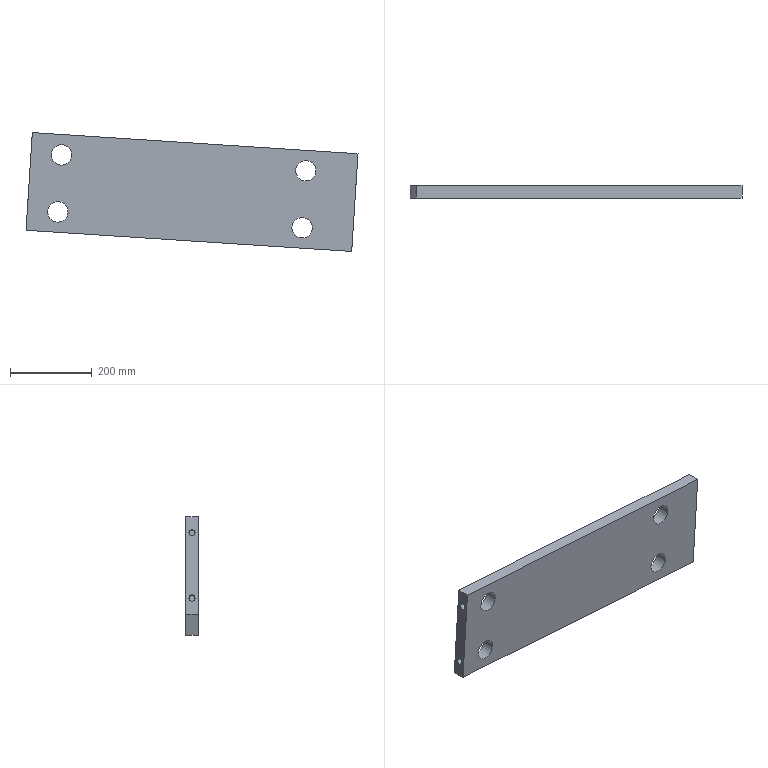Component | SolidWorks | X-AxisPedestal2-3 | 1 solid | 26 faces | box 813.86 x 30 x 291.29 mm | volume 5510243 mm3 | cylinder 16 | plane 10 | commonest cylinder face diameters 15 x8 50 x8
build123d program:
from build123d import *

# Parameters (mm, degrees)
SKETCH1_W               = 800
SKETCH1_H               = 240
BOSS_EXTRUDE1_DEPTH     = 30
CUT_EXTRUDE1_DEPTH      = 887.275
CUT_EXTRUDE1_DEPTH_BACK = 887.275
SKETCH2_R               = 25
SKETCH3_3_R             = 7.5
CUT_EXTRUDE2_DEPTH      = 20
CUT_EXTRUDE3_START      = -780
SKETCH3_3_2_R           = 7.5
CUT_EXTRUDE3_DEPTH      = 20


with BuildPart() as part:
    # Sketch1 → Boss-Extrude1 (new body)
    with BuildSketch(Plane.XY):
        with Locations((-153.487, 571.546)):
            Rectangle(SKETCH1_W, SKETCH1_H)
    extrude(amount=BOSS_EXTRUDE1_DEPTH)

    # Sketch2 → Cut-Extrude1 (cut, two sides: drawn at the far end of the back side and taken through both)
    with BuildSketch(Plane(origin=(0, 0, 0), x_dir=(-1, 0, 0), z_dir=(0, 0, -1)).offset(-CUT_EXTRUDE1_DEPTH_BACK)):
        with Locations((428.487, 501.546)):
            Circle(SKETCH2_R)
        with Locations((428.487, 641.546)):
            Circle(SKETCH2_R)
        with Locations((-171.513, 641.546)):
            Circle(SKETCH2_R)
        with Locations((-171.513, 501.546)):
            Circle(SKETCH2_R)
    extrude(amount=CUT_EXTRUDE1_DEPTH + CUT_EXTRUDE1_DEPTH_BACK, mode=Mode.SUBTRACT)

    # Sketch3_3 → Cut-Extrude2 (cut)
    with BuildSketch(Plane.ZY.offset(553.487)):
        with Locations((15, 651.546)):
            Circle(SKETCH3_3_R)
        with Locations((15, 491.546)):
            Circle(SKETCH3_3_R)
    extrude(amount=-CUT_EXTRUDE2_DEPTH, mode=Mode.SUBTRACT)

    # Sketch3_3 2 → Cut-Extrude3 (cut)
    with BuildSketch(Plane.ZY.offset(553.487).offset(CUT_EXTRUDE3_START)):
        with Locations((15, 651.546)):
            Circle(SKETCH3_3_2_R)
        with Locations((15, 491.546)):
            Circle(SKETCH3_3_2_R)
    extrude(amount=-CUT_EXTRUDE3_DEPTH, mode=Mode.SUBTRACT)


solid = part.part

# Placed as in the assembly
solid = solid.moved(Location((-106.284, -801, 289.801), (90, 0, 176.288)))
STEP:
#1=CARTESIAN_POINT('',(-14.744,-31.831,-13.611));
#2=VERTEX_POINT('',#1);
#3=CARTESIAN_POINT('',(-14.744,-32.421,-13.611));
#4=VERTEX_POINT('',#3);
#5=CARTESIAN_POINT('',(-14.744,-32.126,-13.611));
#6=DIRECTION('',(0.9979,0.,-0.06474));
#7=DIRECTION('',(0.06474,0.,0.9979));
#8=AXIS2_PLACEMENT_3D('',#5,#6,#7);
#9=CIRCLE('',#8,0.2953);
#10=EDGE_CURVE('',#2,#4,#9,.T.);
#11=ORIENTED_EDGE('',*,*,#10,.T.);
#12=CARTESIAN_POINT('',(-15.53,-32.421,-13.56));
#13=VERTEX_POINT('',#12);
#14=CARTESIAN_POINT('',(-14.744,-32.421,-13.611));
#15=DIRECTION('',(-0.9979,-0.,0.06474));
#16=VECTOR('',#15,39.37);
#17=LINE('',#14,#16);
#18=EDGE_CURVE('',#4,#13,#17,.T.);
#19=ORIENTED_EDGE('',*,*,#18,.T.);
#20=CARTESIAN_POINT('',(-15.53,-31.831,-13.56));
#21=VERTEX_POINT('',#20);
#22=CARTESIAN_POINT('',(-15.53,-32.126,-13.56));
#23=DIRECTION('',(0.9979,0.,-0.06474));
#24=DIRECTION('',(0.06474,0.,0.9979));
#25=AXIS2_PLACEMENT_3D('',#22,#23,#24);
#26=CIRCLE('',#25,0.2953);
#27=EDGE_CURVE('',#21,#13,#26,.T.);
#28=ORIENTED_EDGE('',*,*,#27,.F.);
#29=CARTESIAN_POINT('',(-14.744,-31.831,-13.611));
#30=DIRECTION('',(-0.9979,-0.,0.06474));
#31=VECTOR('',#30,39.37);
#32=LINE('',#29,#31);
#33=EDGE_CURVE('',#2,#21,#32,.T.);
#34=ORIENTED_EDGE('',*,*,#33,.F.);
#35=EDGE_LOOP('',(#11,#19,#28,#34));
#36=FACE_OUTER_BOUND('',#35,.T.);
#37=CARTESIAN_POINT('',(-14.744,-32.126,-13.611));
#38=DIRECTION('',(-0.9979,-0.,0.06474));
#39=DIRECTION('',(0.,1.,0.));
#40=AXIS2_PLACEMENT_3D('',#37,#38,#39);
#41=CYLINDRICAL_SURFACE('',#40,0.2953);
#42=ADVANCED_FACE('',(#36),#41,.F.);
#43=CARTESIAN_POINT('',(-14.336,-31.831,-7.325));
#44=VERTEX_POINT('',#43);
#45=CARTESIAN_POINT('',(-14.336,-32.421,-7.325));
#46=VERTEX_POINT('',#45);
#47=CARTESIAN_POINT('',(-14.336,-32.126,-7.325));
#48=DIRECTION('',(0.9979,0.,-0.06474));
#49=DIRECTION('',(0.06474,0.,0.9979));
#50=AXIS2_PLACEMENT_3D('',#47,#48,#49);
#51=CIRCLE('',#50,0.2953);
#52=EDGE_CURVE('',#44,#46,#51,.T.);
#53=ORIENTED_EDGE('',*,*,#52,.T.);
#54=CARTESIAN_POINT('',(-15.122,-32.421,-7.274));
#55=VERTEX_POINT('',#54);
#56=CARTESIAN_POINT('',(-14.336,-32.421,-7.325));
#57=DIRECTION('',(-0.9979,-0.,0.06474));
#58=VECTOR('',#57,39.37);
#59=LINE('',#56,#58);
#60=EDGE_CURVE('',#46,#55,#59,.T.);
#61=ORIENTED_EDGE('',*,*,#60,.T.);
#62=CARTESIAN_POINT('',(-15.122,-31.831,-7.274));
#63=VERTEX_POINT('',#62);
#64=CARTESIAN_POINT('',(-15.122,-32.126,-7.274));
#65=DIRECTION('',(0.9979,0.,-0.06474));
#66=DIRECTION('',(0.06474,0.,0.9979));
#67=AXIS2_PLACEMENT_3D('',#64,#65,#66);
#68=CIRCLE('',#67,0.2953);
#69=EDGE_CURVE('',#63,#55,#68,.T.);
#70=ORIENTED_EDGE('',*,*,#69,.F.);
#71=CARTESIAN_POINT('',(-14.336,-31.831,-7.325));
#72=DIRECTION('',(-0.9979,-0.,0.06474));
#73=VECTOR('',#72,39.37);
#74=LINE('',#71,#73);
#75=EDGE_CURVE('',#44,#63,#74,.T.);
#76=ORIENTED_EDGE('',*,*,#75,.F.);
#77=EDGE_LOOP('',(#53,#61,#70,#76));
#78=FACE_OUTER_BOUND('',#77,.T.);
#79=CARTESIAN_POINT('',(-14.336,-32.126,-7.325));
#80=DIRECTION('',(-0.9979,-0.,0.06474));
#81=DIRECTION('',(0.,1.,0.));
#82=AXIS2_PLACEMENT_3D('',#79,#80,#81);
#83=CYLINDRICAL_SURFACE('',#82,0.2953);
#84=ADVANCED_FACE('',(#78),#83,.F.);
#85=CARTESIAN_POINT('',(15.522,-31.831,-9.262));
#86=VERTEX_POINT('',#85);
#87=CARTESIAN_POINT('',(15.522,-32.421,-9.262));
#88=VERTEX_POINT('',#87);
#89=CARTESIAN_POINT('',(15.522,-32.126,-9.262));
#90=DIRECTION('',(0.9979,0.,-0.06474));
#91=DIRECTION('',(0.,-1.,0.));
#92=AXIS2_PLACEMENT_3D('',#89,#90,#91);
#93=CIRCLE('',#92,0.2953);
#94=EDGE_CURVE('',#86,#88,#93,.T.);
#95=ORIENTED_EDGE('',*,*,#94,.F.);
#96=CARTESIAN_POINT('',(16.308,-31.831,-9.313));
#97=VERTEX_POINT('',#96);
#98=CARTESIAN_POINT('',(15.522,-31.831,-9.262));
#99=DIRECTION('',(0.9979,0.,-0.06474));
#100=VECTOR('',#99,39.37);
#101=LINE('',#98,#100);
#102=EDGE_CURVE('',#86,#97,#101,.T.);
#103=ORIENTED_EDGE('',*,*,#102,.T.);
#104=CARTESIAN_POINT('',(16.308,-32.421,-9.313));
#105=VERTEX_POINT('',#104);
#106=CARTESIAN_POINT('',(16.308,-32.126,-9.313));
#107=DIRECTION('',(0.9979,0.,-0.06474));
#108=DIRECTION('',(0.,-1.,0.));
#109=AXIS2_PLACEMENT_3D('',#106,#107,#108);
#110=CIRCLE('',#109,0.2953);
#111=EDGE_CURVE('',#97,#105,#110,.T.);
#112=ORIENTED_EDGE('',*,*,#111,.T.);
#113=CARTESIAN_POINT('',(15.522,-32.421,-9.262));
#114=DIRECTION('',(0.9979,0.,-0.06474));
#115=VECTOR('',#114,39.37);
#116=LINE('',#113,#115);
#117=EDGE_CURVE('',#88,#105,#116,.T.);
#118=ORIENTED_EDGE('',*,*,#117,.F.);
#119=EDGE_LOOP('',(#95,#103,#112,#118));
#120=FACE_OUTER_BOUND('',#119,.T.);
#121=CARTESIAN_POINT('',(15.522,-32.126,-9.262));
#122=DIRECTION('',(0.9979,0.,-0.06474));
#123=DIRECTION('',(0.,-1.,0.));
#124=AXIS2_PLACEMENT_3D('',#121,#122,#123);
#125=CYLINDRICAL_SURFACE('',#124,0.2953);
#126=ADVANCED_FACE('',(#120),#125,.F.);
#127=CARTESIAN_POINT('',(15.114,-31.831,-15.548));
#128=VERTEX_POINT('',#127);
#129=CARTESIAN_POINT('',(15.114,-32.421,-15.548));
#130=VERTEX_POINT('',#129);
#131=CARTESIAN_POINT('',(15.114,-32.126,-15.548));
#132=DIRECTION('',(0.9979,0.,-0.06474));
#133=DIRECTION('',(0.,-1.,0.));
#134=AXIS2_PLACEMENT_3D('',#131,#132,#133);
#135=CIRCLE('',#134,0.2953);
#136=EDGE_CURVE('',#128,#130,#135,.T.);
#137=ORIENTED_EDGE('',*,*,#136,.F.);
#138=CARTESIAN_POINT('',(15.9,-31.831,-15.599));
#139=VERTEX_POINT('',#138);
#140=CARTESIAN_POINT('',(15.114,-31.831,-15.548));
#141=DIRECTION('',(0.9979,0.,-0.06474));
#142=VECTOR('',#141,39.37);
#143=LINE('',#140,#142);
#144=EDGE_CURVE('',#128,#139,#143,.T.);
#145=ORIENTED_EDGE('',*,*,#144,.T.);
#146=CARTESIAN_POINT('',(15.9,-32.421,-15.599));
#147=VERTEX_POINT('',#146);
#148=CARTESIAN_POINT('',(15.9,-32.126,-15.599));
#149=DIRECTION('',(0.9979,0.,-0.06474));
#150=DIRECTION('',(0.,-1.,0.));
#151=AXIS2_PLACEMENT_3D('',#148,#149,#150);
#152=CIRCLE('',#151,0.2953);
#153=EDGE_CURVE('',#139,#147,#152,.T.);
#154=ORIENTED_EDGE('',*,*,#153,.T.);
#155=CARTESIAN_POINT('',(15.114,-32.421,-15.548));
#156=DIRECTION('',(0.9979,0.,-0.06474));
#157=VECTOR('',#156,39.37);
#158=LINE('',#155,#157);
#159=EDGE_CURVE('',#130,#147,#158,.T.);
#160=ORIENTED_EDGE('',*,*,#159,.F.);
#161=EDGE_LOOP('',(#137,#145,#154,#160));
#162=FACE_OUTER_BOUND('',#161,.T.);
#163=CARTESIAN_POINT('',(15.114,-32.126,-15.548));
#164=DIRECTION('',(0.9979,0.,-0.06474));
#165=DIRECTION('',(0.,-1.,0.));
#166=AXIS2_PLACEMENT_3D('',#163,#164,#165);
#167=CYLINDRICAL_SURFACE('',#166,0.2953);
#168=ADVANCED_FACE('',(#162),#167,.F.);
#169=CARTESIAN_POINT('',(-13.183,-32.717,-7.794));
#170=VERTEX_POINT('',#169);
#171=CARTESIAN_POINT('',(-11.219,-32.717,-7.922));
#172=VERTEX_POINT('',#171);
#173=CARTESIAN_POINT('',(-12.201,-32.717,-7.858));
#174=DIRECTION('',(-0.,1.,0.));
#175=DIRECTION('',(0.9979,0.,-0.06474));
#176=AXIS2_PLACEMENT_3D('',#173,#174,#175);
#177=CIRCLE('',#176,0.9843);
#178=EDGE_CURVE('',#170,#172,#177,.T.);
#179=ORIENTED_EDGE('',*,*,#178,.F.);
#180=CARTESIAN_POINT('',(-13.183,-31.535,-7.794));
#181=VERTEX_POINT('',#180);
#182=CARTESIAN_POINT('',(-13.183,-32.717,-7.794));
#183=DIRECTION('',(-0.,1.,0.));
#184=VECTOR('',#183,39.37);
#185=LINE('',#182,#184);
#186=EDGE_CURVE('',#170,#181,#185,.T.);
#187=ORIENTED_EDGE('',*,*,#186,.T.);
#188=CARTESIAN_POINT('',(-11.219,-31.535,-7.922));
#189=VERTEX_POINT('',#188);
#190=CARTESIAN_POINT('',(-12.201,-31.535,-7.858));
#191=DIRECTION('',(-0.,1.,0.));
#192=DIRECTION('',(0.9979,0.,-0.06474));
#193=AXIS2_PLACEMENT_3D('',#190,#191,#192);
#194=CIRCLE('',#193,0.9843);
#195=EDGE_CURVE('',#181,#189,#194,.T.);
#196=ORIENTED_EDGE('',*,*,#195,.T.);
#197=CARTESIAN_POINT('',(-11.219,-32.717,-7.922));
#198=DIRECTION('',(-0.,1.,0.));
#199=VECTOR('',#198,39.37);
#200=LINE('',#197,#199);
#201=EDGE_CURVE('',#172,#189,#200,.T.);
#202=ORIENTED_EDGE('',*,*,#201,.F.);
#203=EDGE_LOOP('',(#179,#187,#196,#202));
#204=FACE_OUTER_BOUND('',#203,.T.);
#205=CARTESIAN_POINT('',(-12.201,-32.717,-7.858));
#206=DIRECTION('',(-0.,1.,0.));
#207=DIRECTION('',(0.9979,0.,-0.06474));
#208=AXIS2_PLACEMENT_3D('',#205,#206,#207);
#209=CYLINDRICAL_SURFACE('',#208,0.9843);
#210=ADVANCED_FACE('',(#204),#209,.F.);
#211=CARTESIAN_POINT('',(-13.54,-32.717,-13.294));
#212=VERTEX_POINT('',#211);
#213=CARTESIAN_POINT('',(-11.576,-32.717,-13.422));
#214=VERTEX_POINT('',#213);
#215=CARTESIAN_POINT('',(-12.558,-32.717,-13.358));
#216=DIRECTION('',(-0.,1.,0.));
#217=DIRECTION('',(0.9979,0.,-0.06474));
#218=AXIS2_PLACEMENT_3D('',#215,#216,#217);
#219=CIRCLE('',#218,0.9843);
#220=EDGE_CURVE('',#212,#214,#219,.T.);
#221=ORIENTED_EDGE('',*,*,#220,.F.);
#222=CARTESIAN_POINT('',(-13.54,-31.535,-13.294));
#223=VERTEX_POINT('',#222);
#224=CARTESIAN_POINT('',(-13.54,-32.717,-13.294));
#225=DIRECTION('',(-0.,1.,0.));
#226=VECTOR('',#225,39.37);
#227=LINE('',#224,#226);
#228=EDGE_CURVE('',#212,#223,#227,.T.);
#229=ORIENTED_EDGE('',*,*,#228,.T.);
#230=CARTESIAN_POINT('',(-11.576,-31.535,-13.422));
#231=VERTEX_POINT('',#230);
#232=CARTESIAN_POINT('',(-12.558,-31.535,-13.358));
#233=DIRECTION('',(-0.,1.,0.));
#234=DIRECTION('',(0.9979,0.,-0.06474));
#235=AXIS2_PLACEMENT_3D('',#232,#233,#234);
#236=CIRCLE('',#235,0.9843);
#237=EDGE_CURVE('',#223,#231,#236,.T.);
#238=ORIENTED_EDGE('',*,*,#237,.T.);
#239=CARTESIAN_POINT('',(-11.576,-32.717,-13.422));
#240=DIRECTION('',(-0.,1.,0.));
#241=VECTOR('',#240,39.37);
#242=LINE('',#239,#241);
#243=EDGE_CURVE('',#214,#231,#242,.T.);
#244=ORIENTED_EDGE('',*,*,#243,.F.);
#245=EDGE_LOOP('',(#221,#229,#238,#244));
#246=FACE_OUTER_BOUND('',#245,.T.);
#247=CARTESIAN_POINT('',(-12.558,-32.717,-13.358));
#248=DIRECTION('',(-0.,1.,0.));
#249=DIRECTION('',(0.9979,0.,-0.06474));
#250=AXIS2_PLACEMENT_3D('',#247,#248,#249);
#251=CYLINDRICAL_SURFACE('',#250,0.9843);
#252=ADVANCED_FACE('',(#246),#251,.F.);
#253=CARTESIAN_POINT('',(10.032,-32.717,-14.824));
#254=VERTEX_POINT('',#253);
#255=CARTESIAN_POINT('',(11.997,-32.717,-14.951));
#256=VERTEX_POINT('',#255);
#257=CARTESIAN_POINT('',(11.015,-32.717,-14.887));
#258=DIRECTION('',(-0.,1.,0.));
#259=DIRECTION('',(0.9979,0.,-0.06474));
#260=AXIS2_PLACEMENT_3D('',#257,#258,#259);
#261=CIRCLE('',#260,0.9843);
#262=EDGE_CURVE('',#254,#256,#261,.T.);
#263=ORIENTED_EDGE('',*,*,#262,.F.);
#264=CARTESIAN_POINT('',(10.032,-31.535,-14.824));
#265=VERTEX_POINT('',#264);
#266=CARTESIAN_POINT('',(10.032,-32.717,-14.824));
#267=DIRECTION('',(-0.,1.,0.));
#268=VECTOR('',#267,39.37);
#269=LINE('',#266,#268);
#270=EDGE_CURVE('',#254,#265,#269,.T.);
#271=ORIENTED_EDGE('',*,*,#270,.T.);
#272=CARTESIAN_POINT('',(11.997,-31.535,-14.951));
#273=VERTEX_POINT('',#272);
#274=CARTESIAN_POINT('',(11.015,-31.535,-14.887));
#275=DIRECTION('',(-0.,1.,0.));
#276=DIRECTION('',(0.9979,0.,-0.06474));
#277=AXIS2_PLACEMENT_3D('',#274,#275,#276);
#278=CIRCLE('',#277,0.9843);
#279=EDGE_CURVE('',#265,#273,#278,.T.);
#280=ORIENTED_EDGE('',*,*,#279,.T.);
#281=CARTESIAN_POINT('',(11.997,-32.717,-14.951));
#282=DIRECTION('',(-0.,1.,0.));
#283=VECTOR('',#282,39.37);
#284=LINE('',#281,#283);
#285=EDGE_CURVE('',#256,#273,#284,.T.);
#286=ORIENTED_EDGE('',*,*,#285,.F.);
#287=EDGE_LOOP('',(#263,#271,#280,#286));
#288=FACE_OUTER_BOUND('',#287,.T.);
#289=CARTESIAN_POINT('',(11.015,-32.717,-14.887));
#290=DIRECTION('',(-0.,1.,0.));
#291=DIRECTION('',(0.9979,0.,-0.06474));
#292=AXIS2_PLACEMENT_3D('',#289,#290,#291);
#293=CYLINDRICAL_SURFACE('',#292,0.9843);
#294=ADVANCED_FACE('',(#288),#293,.F.);
#295=CARTESIAN_POINT('',(10.389,-32.717,-9.323));
#296=VERTEX_POINT('',#295);
#297=CARTESIAN_POINT('',(12.354,-32.717,-9.451));
#298=VERTEX_POINT('',#297);
#299=CARTESIAN_POINT('',(11.371,-32.717,-9.387));
#300=DIRECTION('',(-0.,1.,0.));
#301=DIRECTION('',(0.9979,0.,-0.06474));
#302=AXIS2_PLACEMENT_3D('',#299,#300,#301);
#303=CIRCLE('',#302,0.9843);
#304=EDGE_CURVE('',#296,#298,#303,.T.);
#305=ORIENTED_EDGE('',*,*,#304,.F.);
#306=CARTESIAN_POINT('',(10.389,-31.535,-9.323));
#307=VERTEX_POINT('',#306);
#308=CARTESIAN_POINT('',(10.389,-32.717,-9.323));
#309=DIRECTION('',(-0.,1.,0.));
#310=VECTOR('',#309,39.37);
#311=LINE('',#308,#310);
#312=EDGE_CURVE('',#296,#307,#311,.T.);
#313=ORIENTED_EDGE('',*,*,#312,.T.);
#314=CARTESIAN_POINT('',(12.354,-31.535,-9.451));
#315=VERTEX_POINT('',#314);
#316=CARTESIAN_POINT('',(11.371,-31.535,-9.387));
#317=DIRECTION('',(-0.,1.,0.));
#318=DIRECTION('',(0.9979,0.,-0.06474));
#319=AXIS2_PLACEMENT_3D('',#316,#317,#318);
#320=CIRCLE('',#319,0.9843);
#321=EDGE_CURVE('',#307,#315,#320,.T.);
#322=ORIENTED_EDGE('',*,*,#321,.T.);
#323=CARTESIAN_POINT('',(12.354,-32.717,-9.451));
#324=DIRECTION('',(-0.,1.,0.));
#325=VECTOR('',#324,39.37);
#326=LINE('',#323,#325);
#327=EDGE_CURVE('',#298,#315,#326,.T.);
#328=ORIENTED_EDGE('',*,*,#327,.F.);
#329=EDGE_LOOP('',(#305,#313,#322,#328));
#330=FACE_OUTER_BOUND('',#329,.T.);
#331=CARTESIAN_POINT('',(11.371,-32.717,-9.387));
#332=DIRECTION('',(-0.,1.,0.));
#333=DIRECTION('',(0.9979,0.,-0.06474));
#334=AXIS2_PLACEMENT_3D('',#331,#332,#333);
#335=CYLINDRICAL_SURFACE('',#334,0.9843);
#336=ADVANCED_FACE('',(#330),#335,.F.);
#337=ORIENTED_EDGE('',*,*,#27,.T.);
#338=CARTESIAN_POINT('',(-15.53,-32.126,-13.56));
#339=DIRECTION('',(0.9979,0.,-0.06474));
#340=DIRECTION('',(0.06474,0.,0.9979));
#341=AXIS2_PLACEMENT_3D('',#338,#339,#340);
#342=CIRCLE('',#341,0.2953);
#343=EDGE_CURVE('',#13,#21,#342,.T.);
#344=ORIENTED_EDGE('',*,*,#343,.T.);
#345=EDGE_LOOP('',(#337,#344));
#346=FACE_BOUND('',#345,.T.);
#347=ORIENTED_EDGE('',*,*,#69,.T.);
#348=CARTESIAN_POINT('',(-15.122,-32.126,-7.274));
#349=DIRECTION('',(0.9979,0.,-0.06474));
#350=DIRECTION('',(0.06474,0.,0.9979));
#351=AXIS2_PLACEMENT_3D('',#348,#349,#350);
#352=CIRCLE('',#351,0.2953);
#353=EDGE_CURVE('',#55,#63,#352,.T.);
#354=ORIENTED_EDGE('',*,*,#353,.T.);
#355=EDGE_LOOP('',(#347,#354));
#356=FACE_BOUND('',#355,.T.);
#357=CARTESIAN_POINT('',(-15.02,-31.535,-5.702));
#358=VERTEX_POINT('',#357);
#359=CARTESIAN_POINT('',(-15.632,-31.535,-15.131));
#360=VERTEX_POINT('',#359);
#361=CARTESIAN_POINT('',(-15.632,-31.535,-15.131));
#362=DIRECTION('',(-0.06474,0.,-0.9979));
#363=VECTOR('',#362,39.37);
#364=LINE('',#361,#363);
#365=EDGE_CURVE('',#358,#360,#364,.T.);
#366=ORIENTED_EDGE('',*,*,#365,.T.);
#367=CARTESIAN_POINT('',(-15.632,-32.717,-15.131));
#368=VERTEX_POINT('',#367);
#369=CARTESIAN_POINT('',(-15.632,-32.717,-15.131));
#370=DIRECTION('',(-0.,1.,0.));
#371=VECTOR('',#370,39.37);
#372=LINE('',#369,#371);
#373=EDGE_CURVE('',#368,#360,#372,.T.);
#374=ORIENTED_EDGE('',*,*,#373,.F.);
#375=CARTESIAN_POINT('',(-15.02,-32.717,-5.702));
#376=VERTEX_POINT('',#375);
#377=CARTESIAN_POINT('',(-15.632,-32.717,-15.131));
#378=DIRECTION('',(-0.06474,0.,-0.9979));
#379=VECTOR('',#378,39.37);
#380=LINE('',#377,#379);
#381=EDGE_CURVE('',#376,#368,#380,.T.);
#382=ORIENTED_EDGE('',*,*,#381,.F.);
#383=CARTESIAN_POINT('',(-15.02,-32.717,-5.702));
#384=DIRECTION('',(-0.,1.,0.));
#385=VECTOR('',#384,39.37);
#386=LINE('',#383,#385);
#387=EDGE_CURVE('',#376,#358,#386,.T.);
#388=ORIENTED_EDGE('',*,*,#387,.T.);
#389=EDGE_LOOP('',(#366,#374,#382,#388));
#390=FACE_OUTER_BOUND('',#389,.T.);
#391=CARTESIAN_POINT('',(-15.632,-32.717,-15.131));
#392=DIRECTION('',(0.9979,0.,-0.06474));
#393=DIRECTION('',(0.06474,-0.,0.9979));
#394=AXIS2_PLACEMENT_3D('',#391,#392,#393);
#395=PLANE('',#394);
#396=ADVANCED_FACE('',(#346,#356,#390),#395,.F.);
#397=CARTESIAN_POINT('',(15.798,-31.535,-17.17));
#398=VERTEX_POINT('',#397);
#399=CARTESIAN_POINT('',(-15.632,-31.535,-15.131));
#400=DIRECTION('',(0.9979,0.,-0.06474));
#401=VECTOR('',#400,39.37);
#402=LINE('',#399,#401);
#403=EDGE_CURVE('',#360,#398,#402,.T.);
#404=ORIENTED_EDGE('',*,*,#403,.T.);
#405=CARTESIAN_POINT('',(15.798,-32.717,-17.17));
#406=VERTEX_POINT('',#405);
#407=CARTESIAN_POINT('',(15.798,-32.717,-17.17));
#408=DIRECTION('',(-0.,1.,0.));
#409=VECTOR('',#408,39.37);
#410=LINE('',#407,#409);
#411=EDGE_CURVE('',#406,#398,#410,.T.);
#412=ORIENTED_EDGE('',*,*,#411,.F.);
#413=CARTESIAN_POINT('',(-15.632,-32.717,-15.131));
#414=DIRECTION('',(0.9979,0.,-0.06474));
#415=VECTOR('',#414,39.37);
#416=LINE('',#413,#415);
#417=EDGE_CURVE('',#368,#406,#416,.T.);
#418=ORIENTED_EDGE('',*,*,#417,.F.);
#419=ORIENTED_EDGE('',*,*,#373,.T.);
#420=EDGE_LOOP('',(#404,#412,#418,#419));
#421=FACE_OUTER_BOUND('',#420,.T.);
#422=CARTESIAN_POINT('',(-15.632,-32.717,-15.131));
#423=DIRECTION('',(0.06474,-0.,0.9979));
#424=DIRECTION('',(-0.9979,-0.,0.06474));
#425=AXIS2_PLACEMENT_3D('',#422,#423,#424);
#426=PLANE('',#425);
#427=ADVANCED_FACE('',(#421),#426,.F.);
#428=CARTESIAN_POINT('',(16.308,-32.126,-9.313));
#429=DIRECTION('',(0.9979,0.,-0.06474));
#430=DIRECTION('',(0.,-1.,0.));
#431=AXIS2_PLACEMENT_3D('',#428,#429,#430);
#432=CIRCLE('',#431,0.2953);
#433=EDGE_CURVE('',#105,#97,#432,.T.);
#434=ORIENTED_EDGE('',*,*,#433,.F.);
#435=ORIENTED_EDGE('',*,*,#111,.F.);
#436=EDGE_LOOP('',(#434,#435));
#437=FACE_BOUND('',#436,.T.);
#438=CARTESIAN_POINT('',(15.9,-32.126,-15.599));
#439=DIRECTION('',(0.9979,0.,-0.06474));
#440=DIRECTION('',(0.,-1.,0.));
#441=AXIS2_PLACEMENT_3D('',#438,#439,#440);
#442=CIRCLE('',#441,0.2953);
#443=EDGE_CURVE('',#147,#139,#442,.T.);
#444=ORIENTED_EDGE('',*,*,#443,.F.);
#445=ORIENTED_EDGE('',*,*,#153,.F.);
#446=EDGE_LOOP('',(#444,#445));
#447=FACE_BOUND('',#446,.T.);
#448=CARTESIAN_POINT('',(16.41,-31.535,-7.741));
#449=VERTEX_POINT('',#448);
#450=CARTESIAN_POINT('',(15.798,-31.535,-17.17));
#451=DIRECTION('',(0.06474,-0.,0.9979));
#452=VECTOR('',#451,39.37);
#453=LINE('',#450,#452);
#454=EDGE_CURVE('',#398,#449,#453,.T.);
#455=ORIENTED_EDGE('',*,*,#454,.T.);
#456=CARTESIAN_POINT('',(16.41,-32.717,-7.741));
#457=VERTEX_POINT('',#456);
#458=CARTESIAN_POINT('',(16.41,-32.717,-7.741));
#459=DIRECTION('',(-0.,1.,0.));
#460=VECTOR('',#459,39.37);
#461=LINE('',#458,#460);
#462=EDGE_CURVE('',#457,#449,#461,.T.);
#463=ORIENTED_EDGE('',*,*,#462,.F.);
#464=CARTESIAN_POINT('',(15.798,-32.717,-17.17));
#465=DIRECTION('',(0.06474,-0.,0.9979));
#466=VECTOR('',#465,39.37);
#467=LINE('',#464,#466);
#468=EDGE_CURVE('',#406,#457,#467,.T.);
#469=ORIENTED_EDGE('',*,*,#468,.F.);
#470=ORIENTED_EDGE('',*,*,#411,.T.);
#471=EDGE_LOOP('',(#455,#463,#469,#470));
#472=FACE_OUTER_BOUND('',#471,.T.);
#473=CARTESIAN_POINT('',(15.798,-32.717,-17.17));
#474=DIRECTION('',(-0.9979,-0.,0.06474));
#475=DIRECTION('',(-0.,1.,0.));
#476=AXIS2_PLACEMENT_3D('',#473,#474,#475);
#477=PLANE('',#476);
#478=ADVANCED_FACE('',(#437,#447,#472),#477,.F.);
#479=CARTESIAN_POINT('',(-15.02,-31.535,-5.702));
#480=DIRECTION('',(-0.9979,-0.,0.06474));
#481=VECTOR('',#480,39.37);
#482=LINE('',#479,#481);
#483=EDGE_CURVE('',#449,#358,#482,.T.);
#484=ORIENTED_EDGE('',*,*,#483,.T.);
#485=ORIENTED_EDGE('',*,*,#387,.F.);
#486=CARTESIAN_POINT('',(-15.02,-32.717,-5.702));
#487=DIRECTION('',(-0.9979,-0.,0.06474));
#488=VECTOR('',#487,39.37);
#489=LINE('',#486,#488);
#490=EDGE_CURVE('',#457,#376,#489,.T.);
#491=ORIENTED_EDGE('',*,*,#490,.F.);
#492=ORIENTED_EDGE('',*,*,#462,.T.);
#493=EDGE_LOOP('',(#484,#485,#491,#492));
#494=FACE_OUTER_BOUND('',#493,.T.);
#495=CARTESIAN_POINT('',(-15.02,-32.717,-5.702));
#496=DIRECTION('',(-0.06474,0.,-0.9979));
#497=DIRECTION('',(0.9979,0.,-0.06474));
#498=AXIS2_PLACEMENT_3D('',#495,#496,#497);
#499=PLANE('',#498);
#500=ADVANCED_FACE('',(#494),#499,.F.);
#501=CARTESIAN_POINT('',(-12.201,-32.717,-7.858));
#502=DIRECTION('',(-0.,1.,0.));
#503=DIRECTION('',(0.9979,0.,-0.06474));
#504=AXIS2_PLACEMENT_3D('',#501,#502,#503);
#505=CIRCLE('',#504,0.9843);
#506=EDGE_CURVE('',#172,#170,#505,.T.);
#507=ORIENTED_EDGE('',*,*,#506,.T.);
#508=ORIENTED_EDGE('',*,*,#178,.T.);
#509=EDGE_LOOP('',(#507,#508));
#510=FACE_BOUND('',#509,.T.);
#511=CARTESIAN_POINT('',(-12.558,-32.717,-13.358));
#512=DIRECTION('',(-0.,1.,0.));
#513=DIRECTION('',(0.9979,0.,-0.06474));
#514=AXIS2_PLACEMENT_3D('',#511,#512,#513);
#515=CIRCLE('',#514,0.9843);
#516=EDGE_CURVE('',#214,#212,#515,.T.);
#517=ORIENTED_EDGE('',*,*,#516,.T.);
#518=ORIENTED_EDGE('',*,*,#220,.T.);
#519=EDGE_LOOP('',(#517,#518));
#520=FACE_BOUND('',#519,.T.);
#521=CARTESIAN_POINT('',(11.015,-32.717,-14.887));
#522=DIRECTION('',(-0.,1.,0.));
#523=DIRECTION('',(0.9979,0.,-0.06474));
#524=AXIS2_PLACEMENT_3D('',#521,#522,#523);
#525=CIRCLE('',#524,0.9843);
#526=EDGE_CURVE('',#256,#254,#525,.T.);
#527=ORIENTED_EDGE('',*,*,#526,.T.);
#528=ORIENTED_EDGE('',*,*,#262,.T.);
#529=EDGE_LOOP('',(#527,#528));
#530=FACE_BOUND('',#529,.T.);
#531=CARTESIAN_POINT('',(11.371,-32.717,-9.387));
#532=DIRECTION('',(-0.,1.,0.));
#533=DIRECTION('',(0.9979,0.,-0.06474));
#534=AXIS2_PLACEMENT_3D('',#531,#532,#533);
#535=CIRCLE('',#534,0.9843);
#536=EDGE_CURVE('',#298,#296,#535,.T.);
#537=ORIENTED_EDGE('',*,*,#536,.T.);
#538=ORIENTED_EDGE('',*,*,#304,.T.);
#539=EDGE_LOOP('',(#537,#538));
#540=FACE_BOUND('',#539,.T.);
#541=ORIENTED_EDGE('',*,*,#381,.T.);
#542=ORIENTED_EDGE('',*,*,#417,.T.);
#543=ORIENTED_EDGE('',*,*,#468,.T.);
#544=ORIENTED_EDGE('',*,*,#490,.T.);
#545=EDGE_LOOP('',(#541,#542,#543,#544));
#546=FACE_OUTER_BOUND('',#545,.T.);
#547=CARTESIAN_POINT('',(-4.184,-32.717,11.41));
#548=DIRECTION('',(-0.,1.,0.));
#549=DIRECTION('',(0.9979,0.,-0.06474));
#550=AXIS2_PLACEMENT_3D('',#547,#548,#549);
#551=PLANE('',#550);
#552=ADVANCED_FACE('',(#510,#520,#530,#540,#546),#551,.F.);
#553=CARTESIAN_POINT('',(-12.201,-31.535,-7.858));
#554=DIRECTION('',(-0.,1.,0.));
#555=DIRECTION('',(0.9979,0.,-0.06474));
#556=AXIS2_PLACEMENT_3D('',#553,#554,#555);
#557=CIRCLE('',#556,0.9843);
#558=EDGE_CURVE('',#189,#181,#557,.T.);
#559=ORIENTED_EDGE('',*,*,#558,.F.);
#560=ORIENTED_EDGE('',*,*,#195,.F.);
#561=EDGE_LOOP('',(#559,#560));
#562=FACE_BOUND('',#561,.T.);
#563=CARTESIAN_POINT('',(-12.558,-31.535,-13.358));
#564=DIRECTION('',(-0.,1.,0.));
#565=DIRECTION('',(0.9979,0.,-0.06474));
#566=AXIS2_PLACEMENT_3D('',#563,#564,#565);
#567=CIRCLE('',#566,0.9843);
#568=EDGE_CURVE('',#231,#223,#567,.T.);
#569=ORIENTED_EDGE('',*,*,#568,.F.);
#570=ORIENTED_EDGE('',*,*,#237,.F.);
#571=EDGE_LOOP('',(#569,#570));
#572=FACE_BOUND('',#571,.T.);
#573=CARTESIAN_POINT('',(11.015,-31.535,-14.887));
#574=DIRECTION('',(-0.,1.,0.));
#575=DIRECTION('',(0.9979,0.,-0.06474));
#576=AXIS2_PLACEMENT_3D('',#573,#574,#575);
#577=CIRCLE('',#576,0.9843);
#578=EDGE_CURVE('',#273,#265,#577,.T.);
#579=ORIENTED_EDGE('',*,*,#578,.F.);
#580=ORIENTED_EDGE('',*,*,#279,.F.);
#581=EDGE_LOOP('',(#579,#580));
#582=FACE_BOUND('',#581,.T.);
#583=CARTESIAN_POINT('',(11.371,-31.535,-9.387));
#584=DIRECTION('',(-0.,1.,0.));
#585=DIRECTION('',(0.9979,0.,-0.06474));
#586=AXIS2_PLACEMENT_3D('',#583,#584,#585);
#587=CIRCLE('',#586,0.9843);
#588=EDGE_CURVE('',#315,#307,#587,.T.);
#589=ORIENTED_EDGE('',*,*,#588,.F.);
#590=ORIENTED_EDGE('',*,*,#321,.F.);
#591=EDGE_LOOP('',(#589,#590));
#592=FACE_BOUND('',#591,.T.);
#593=ORIENTED_EDGE('',*,*,#365,.F.);
#594=ORIENTED_EDGE('',*,*,#483,.F.);
#595=ORIENTED_EDGE('',*,*,#454,.F.);
#596=ORIENTED_EDGE('',*,*,#403,.F.);
#597=EDGE_LOOP('',(#593,#594,#595,#596));
#598=FACE_OUTER_BOUND('',#597,.T.);
#599=CARTESIAN_POINT('',(-4.184,-31.535,11.41));
#600=DIRECTION('',(-0.,1.,0.));
#601=DIRECTION('',(0.9979,0.,-0.06474));
#602=AXIS2_PLACEMENT_3D('',#599,#600,#601);
#603=PLANE('',#602);
#604=ADVANCED_FACE('',(#562,#572,#582,#592,#598),#603,.T.);
#605=ORIENTED_EDGE('',*,*,#312,.F.);
#606=ORIENTED_EDGE('',*,*,#536,.F.);
#607=ORIENTED_EDGE('',*,*,#327,.T.);
#608=ORIENTED_EDGE('',*,*,#588,.T.);
#609=EDGE_LOOP('',(#605,#606,#607,#608));
#610=FACE_OUTER_BOUND('',#609,.T.);
#611=CARTESIAN_POINT('',(11.371,-32.717,-9.387));
#612=DIRECTION('',(-0.,1.,0.));
#613=DIRECTION('',(0.9979,0.,-0.06474));
#614=AXIS2_PLACEMENT_3D('',#611,#612,#613);
#615=CYLINDRICAL_SURFACE('',#614,0.9843);
#616=ADVANCED_FACE('',(#610),#615,.F.);
#617=ORIENTED_EDGE('',*,*,#270,.F.);
#618=ORIENTED_EDGE('',*,*,#526,.F.);
#619=ORIENTED_EDGE('',*,*,#285,.T.);
#620=ORIENTED_EDGE('',*,*,#578,.T.);
#621=EDGE_LOOP('',(#617,#618,#619,#620));
#622=FACE_OUTER_BOUND('',#621,.T.);
#623=CARTESIAN_POINT('',(11.015,-32.717,-14.887));
#624=DIRECTION('',(-0.,1.,0.));
#625=DIRECTION('',(0.9979,0.,-0.06474));
#626=AXIS2_PLACEMENT_3D('',#623,#624,#625);
#627=CYLINDRICAL_SURFACE('',#626,0.9843);
#628=ADVANCED_FACE('',(#622),#627,.F.);
#629=ORIENTED_EDGE('',*,*,#228,.F.);
#630=ORIENTED_EDGE('',*,*,#516,.F.);
#631=ORIENTED_EDGE('',*,*,#243,.T.);
#632=ORIENTED_EDGE('',*,*,#568,.T.);
#633=EDGE_LOOP('',(#629,#630,#631,#632));
#634=FACE_OUTER_BOUND('',#633,.T.);
#635=CARTESIAN_POINT('',(-12.558,-32.717,-13.358));
#636=DIRECTION('',(-0.,1.,0.));
#637=DIRECTION('',(0.9979,0.,-0.06474));
#638=AXIS2_PLACEMENT_3D('',#635,#636,#637);
#639=CYLINDRICAL_SURFACE('',#638,0.9843);
#640=ADVANCED_FACE('',(#634),#639,.F.);
#641=ORIENTED_EDGE('',*,*,#186,.F.);
#642=ORIENTED_EDGE('',*,*,#506,.F.);
#643=ORIENTED_EDGE('',*,*,#201,.T.);
#644=ORIENTED_EDGE('',*,*,#558,.T.);
#645=EDGE_LOOP('',(#641,#642,#643,#644));
#646=FACE_OUTER_BOUND('',#645,.T.);
#647=CARTESIAN_POINT('',(-12.201,-32.717,-7.858));
#648=DIRECTION('',(-0.,1.,0.));
#649=DIRECTION('',(0.9979,0.,-0.06474));
#650=AXIS2_PLACEMENT_3D('',#647,#648,#649);
#651=CYLINDRICAL_SURFACE('',#650,0.9843);
#652=ADVANCED_FACE('',(#646),#651,.F.);
#653=ORIENTED_EDGE('',*,*,#144,.F.);
#654=CARTESIAN_POINT('',(15.114,-32.126,-15.548));
#655=DIRECTION('',(0.9979,0.,-0.06474));
#656=DIRECTION('',(0.,-1.,0.));
#657=AXIS2_PLACEMENT_3D('',#654,#655,#656);
#658=CIRCLE('',#657,0.2953);
#659=EDGE_CURVE('',#130,#128,#658,.T.);
#660=ORIENTED_EDGE('',*,*,#659,.F.);
#661=ORIENTED_EDGE('',*,*,#159,.T.);
#662=ORIENTED_EDGE('',*,*,#443,.T.);
#663=EDGE_LOOP('',(#653,#660,#661,#662));
#664=FACE_OUTER_BOUND('',#663,.T.);
#665=CARTESIAN_POINT('',(15.114,-32.126,-15.548));
#666=DIRECTION('',(0.9979,0.,-0.06474));
#667=DIRECTION('',(0.,-1.,0.));
#668=AXIS2_PLACEMENT_3D('',#665,#666,#667);
#669=CYLINDRICAL_SURFACE('',#668,0.2953);
#670=ADVANCED_FACE('',(#664),#669,.F.);
#671=ORIENTED_EDGE('',*,*,#659,.T.);
#672=ORIENTED_EDGE('',*,*,#136,.T.);
#673=EDGE_LOOP('',(#671,#672));
#674=FACE_OUTER_BOUND('',#673,.T.);
#675=CARTESIAN_POINT('',(15.114,-32.126,-15.548));
#676=DIRECTION('',(0.9979,0.,-0.06474));
#677=DIRECTION('',(0.,-1.,-0.));
#678=AXIS2_PLACEMENT_3D('',#675,#676,#677);
#679=PLANE('',#678);
#680=ADVANCED_FACE('',(#674),#679,.T.);
#681=ORIENTED_EDGE('',*,*,#102,.F.);
#682=CARTESIAN_POINT('',(15.522,-32.126,-9.262));
#683=DIRECTION('',(0.9979,0.,-0.06474));
#684=DIRECTION('',(0.,-1.,0.));
#685=AXIS2_PLACEMENT_3D('',#682,#683,#684);
#686=CIRCLE('',#685,0.2953);
#687=EDGE_CURVE('',#88,#86,#686,.T.);
#688=ORIENTED_EDGE('',*,*,#687,.F.);
#689=ORIENTED_EDGE('',*,*,#117,.T.);
#690=ORIENTED_EDGE('',*,*,#433,.T.);
#691=EDGE_LOOP('',(#681,#688,#689,#690));
#692=FACE_OUTER_BOUND('',#691,.T.);
#693=CARTESIAN_POINT('',(15.522,-32.126,-9.262));
#694=DIRECTION('',(0.9979,0.,-0.06474));
#695=DIRECTION('',(0.,-1.,0.));
#696=AXIS2_PLACEMENT_3D('',#693,#694,#695);
#697=CYLINDRICAL_SURFACE('',#696,0.2953);
#698=ADVANCED_FACE('',(#692),#697,.F.);
#699=ORIENTED_EDGE('',*,*,#687,.T.);
#700=ORIENTED_EDGE('',*,*,#94,.T.);
#701=EDGE_LOOP('',(#699,#700));
#702=FACE_OUTER_BOUND('',#701,.T.);
#703=CARTESIAN_POINT('',(15.522,-32.126,-9.262));
#704=DIRECTION('',(0.9979,0.,-0.06474));
#705=DIRECTION('',(0.,-1.,-0.));
#706=AXIS2_PLACEMENT_3D('',#703,#704,#705);
#707=PLANE('',#706);
#708=ADVANCED_FACE('',(#702),#707,.T.);
#709=ORIENTED_EDGE('',*,*,#60,.F.);
#710=CARTESIAN_POINT('',(-14.336,-32.126,-7.325));
#711=DIRECTION('',(0.9979,0.,-0.06474));
#712=DIRECTION('',(0.06474,0.,0.9979));
#713=AXIS2_PLACEMENT_3D('',#710,#711,#712);
#714=CIRCLE('',#713,0.2953);
#715=EDGE_CURVE('',#46,#44,#714,.T.);
#716=ORIENTED_EDGE('',*,*,#715,.T.);
#717=ORIENTED_EDGE('',*,*,#75,.T.);
#718=ORIENTED_EDGE('',*,*,#353,.F.);
#719=EDGE_LOOP('',(#709,#716,#717,#718));
#720=FACE_OUTER_BOUND('',#719,.T.);
#721=CARTESIAN_POINT('',(-14.336,-32.126,-7.325));
#722=DIRECTION('',(-0.9979,-0.,0.06474));
#723=DIRECTION('',(0.,1.,0.));
#724=AXIS2_PLACEMENT_3D('',#721,#722,#723);
#725=CYLINDRICAL_SURFACE('',#724,0.2953);
#726=ADVANCED_FACE('',(#720),#725,.F.);
#727=ORIENTED_EDGE('',*,*,#52,.F.);
#728=ORIENTED_EDGE('',*,*,#715,.F.);
#729=EDGE_LOOP('',(#727,#728));
#730=FACE_OUTER_BOUND('',#729,.T.);
#731=CARTESIAN_POINT('',(-14.336,-32.126,-7.325));
#732=DIRECTION('',(0.9979,0.,-0.06474));
#733=DIRECTION('',(0.06474,-0.,0.9979));
#734=AXIS2_PLACEMENT_3D('',#731,#732,#733);
#735=PLANE('',#734);
#736=ADVANCED_FACE('',(#730),#735,.F.);
#737=ORIENTED_EDGE('',*,*,#18,.F.);
#738=CARTESIAN_POINT('',(-14.744,-32.126,-13.611));
#739=DIRECTION('',(0.9979,0.,-0.06474));
#740=DIRECTION('',(0.06474,0.,0.9979));
#741=AXIS2_PLACEMENT_3D('',#738,#739,#740);
#742=CIRCLE('',#741,0.2953);
#743=EDGE_CURVE('',#4,#2,#742,.T.);
#744=ORIENTED_EDGE('',*,*,#743,.T.);
#745=ORIENTED_EDGE('',*,*,#33,.T.);
#746=ORIENTED_EDGE('',*,*,#343,.F.);
#747=EDGE_LOOP('',(#737,#744,#745,#746));
#748=FACE_OUTER_BOUND('',#747,.T.);
#749=CARTESIAN_POINT('',(-14.744,-32.126,-13.611));
#750=DIRECTION('',(-0.9979,-0.,0.06474));
#751=DIRECTION('',(0.,1.,0.));
#752=AXIS2_PLACEMENT_3D('',#749,#750,#751);
#753=CYLINDRICAL_SURFACE('',#752,0.2953);
#754=ADVANCED_FACE('',(#748),#753,.F.);
#755=ORIENTED_EDGE('',*,*,#10,.F.);
#756=ORIENTED_EDGE('',*,*,#743,.F.);
#757=EDGE_LOOP('',(#755,#756));
#758=FACE_OUTER_BOUND('',#757,.T.);
#759=CARTESIAN_POINT('',(-14.744,-32.126,-13.611));
#760=DIRECTION('',(0.9979,0.,-0.06474));
#761=DIRECTION('',(0.06474,-0.,0.9979));
#762=AXIS2_PLACEMENT_3D('',#759,#760,#761);
#763=PLANE('',#762);
#764=ADVANCED_FACE('',(#758),#763,.F.);
#765=CLOSED_SHELL('',(#42,#84,#126,#168,#210,#252,#294,#336,#396,#427,#478,#500,#552,#604,#616,#628,#640,#652,#670,#680,#698,#708,#726,#736,#754,#764));
#766=MANIFOLD_SOLID_BREP('',#765);
#767=CARTESIAN_POINT('',(0.,0.,0.));
#768=DIRECTION('',(0.,0.,1.));
#769=DIRECTION('',(1.,0.,0.));
#770=AXIS2_PLACEMENT_3D('',#767,#768,#769);
#771=(LENGTH_UNIT()NAMED_UNIT(*)SI_UNIT($,.METRE.));
#772=LENGTH_MEASURE_WITH_UNIT(LENGTH_MEASURE(0.0254),#771);
#773=DIMENSIONAL_EXPONENTS(1.,0.,0.,0.,0.,0.,0.);
#774=(CONVERSION_BASED_UNIT('',#772)LENGTH_UNIT()NAMED_UNIT(#773));
#775=UNCERTAINTY_MEASURE_WITH_UNIT(LENGTH_MEASURE(0.00001),#774,'','');
#776=(NAMED_UNIT(*)PLANE_ANGLE_UNIT()SI_UNIT($,.RADIAN.));
#777=(NAMED_UNIT(*)SI_UNIT($,.STERADIAN.)SOLID_ANGLE_UNIT());
#778=(GEOMETRIC_REPRESENTATION_CONTEXT(3)GLOBAL_UNCERTAINTY_ASSIGNED_CONTEXT((#775))GLOBAL_UNIT_ASSIGNED_CONTEXT((#774,#776,#777))REPRESENTATION_CONTEXT('',''));
#779=ADVANCED_BREP_SHAPE_REPRESENTATION('',(#766,#770),#778);
#780=COLOUR_RGB('',0.7922,0.8196,0.9333);
#781=FILL_AREA_STYLE_COLOUR('',#780);
#782=FILL_AREA_STYLE('',(#781));
#783=SURFACE_STYLE_FILL_AREA(#782);
#784=SURFACE_SIDE_STYLE('',(#783));
#785=SURFACE_STYLE_USAGE(.BOTH.,#784);
#786=PRESENTATION_STYLE_ASSIGNMENT((#785));
#787=STYLED_ITEM('',(#786),#766);
#788=PRESENTATION_LAYER_ASSIGNMENT('','',(#787));
#789=(LENGTH_UNIT()NAMED_UNIT(*)SI_UNIT($,.METRE.));
#790=LENGTH_MEASURE_WITH_UNIT(LENGTH_MEASURE(0.0254),#789);
#791=DIMENSIONAL_EXPONENTS(1.,0.,0.,0.,0.,0.,0.);
#792=(CONVERSION_BASED_UNIT('',#790)LENGTH_UNIT()NAMED_UNIT(#791));
#793=UNCERTAINTY_MEASURE_WITH_UNIT(LENGTH_MEASURE(0.00001),#792,'','');
#794=(NAMED_UNIT(*)PLANE_ANGLE_UNIT()SI_UNIT($,.RADIAN.));
#795=(NAMED_UNIT(*)SI_UNIT($,.STERADIAN.)SOLID_ANGLE_UNIT());
#796=(GEOMETRIC_REPRESENTATION_CONTEXT(3)GLOBAL_UNCERTAINTY_ASSIGNED_CONTEXT((#793))GLOBAL_UNIT_ASSIGNED_CONTEXT((#792,#794,#795))REPRESENTATION_CONTEXT('',''));
#797=MECHANICAL_DESIGN_GEOMETRIC_PRESENTATION_REPRESENTATION('',(#787),#796);